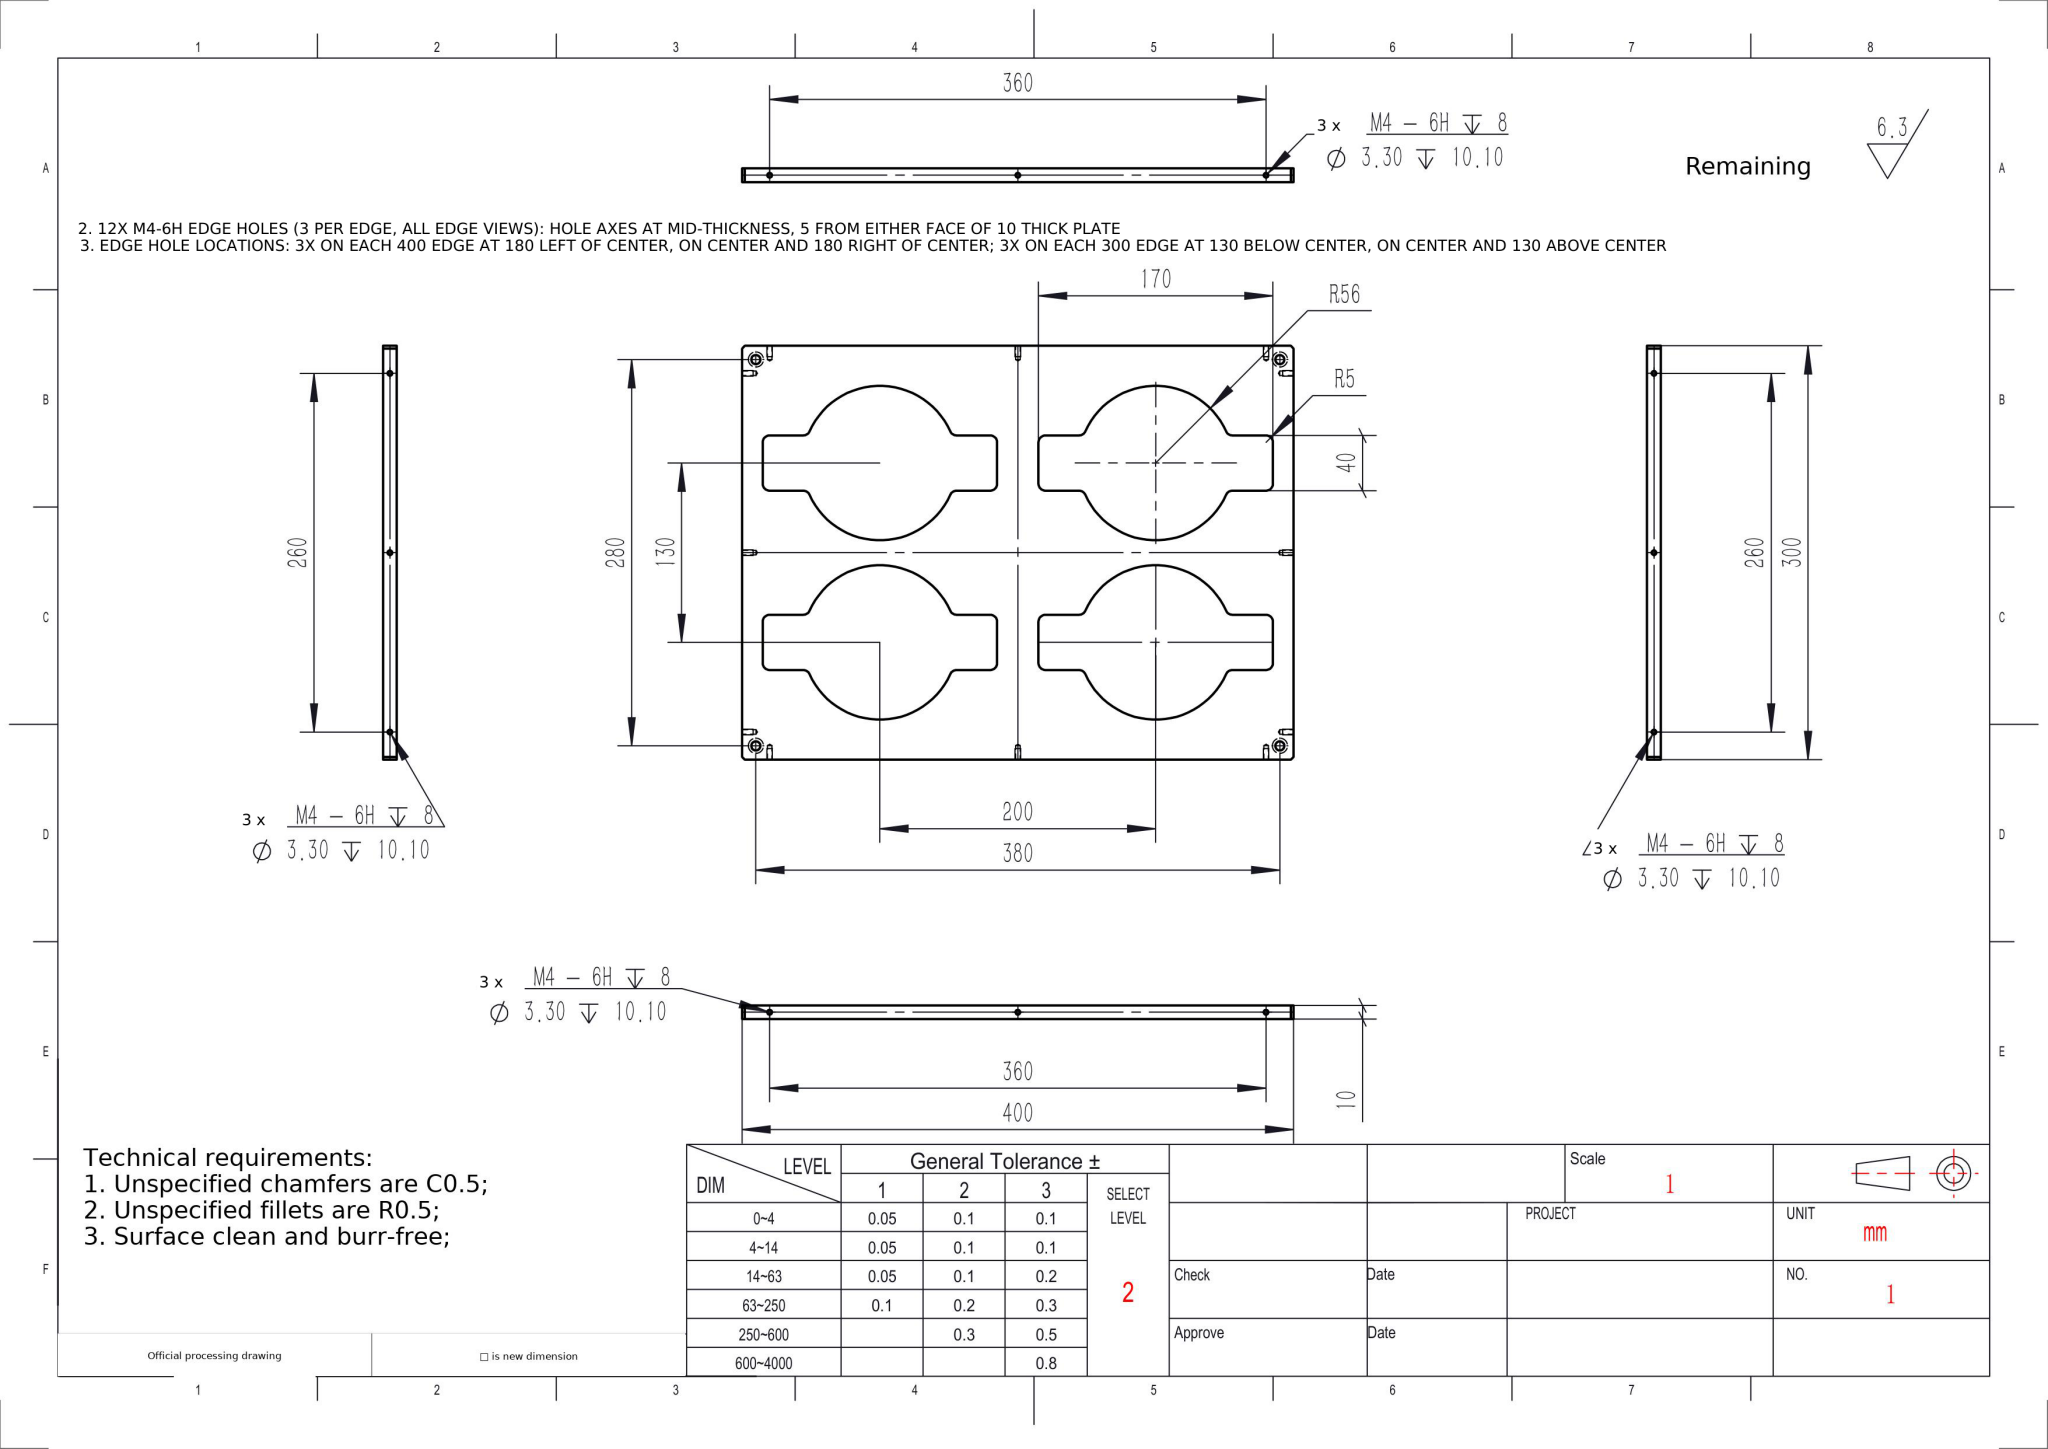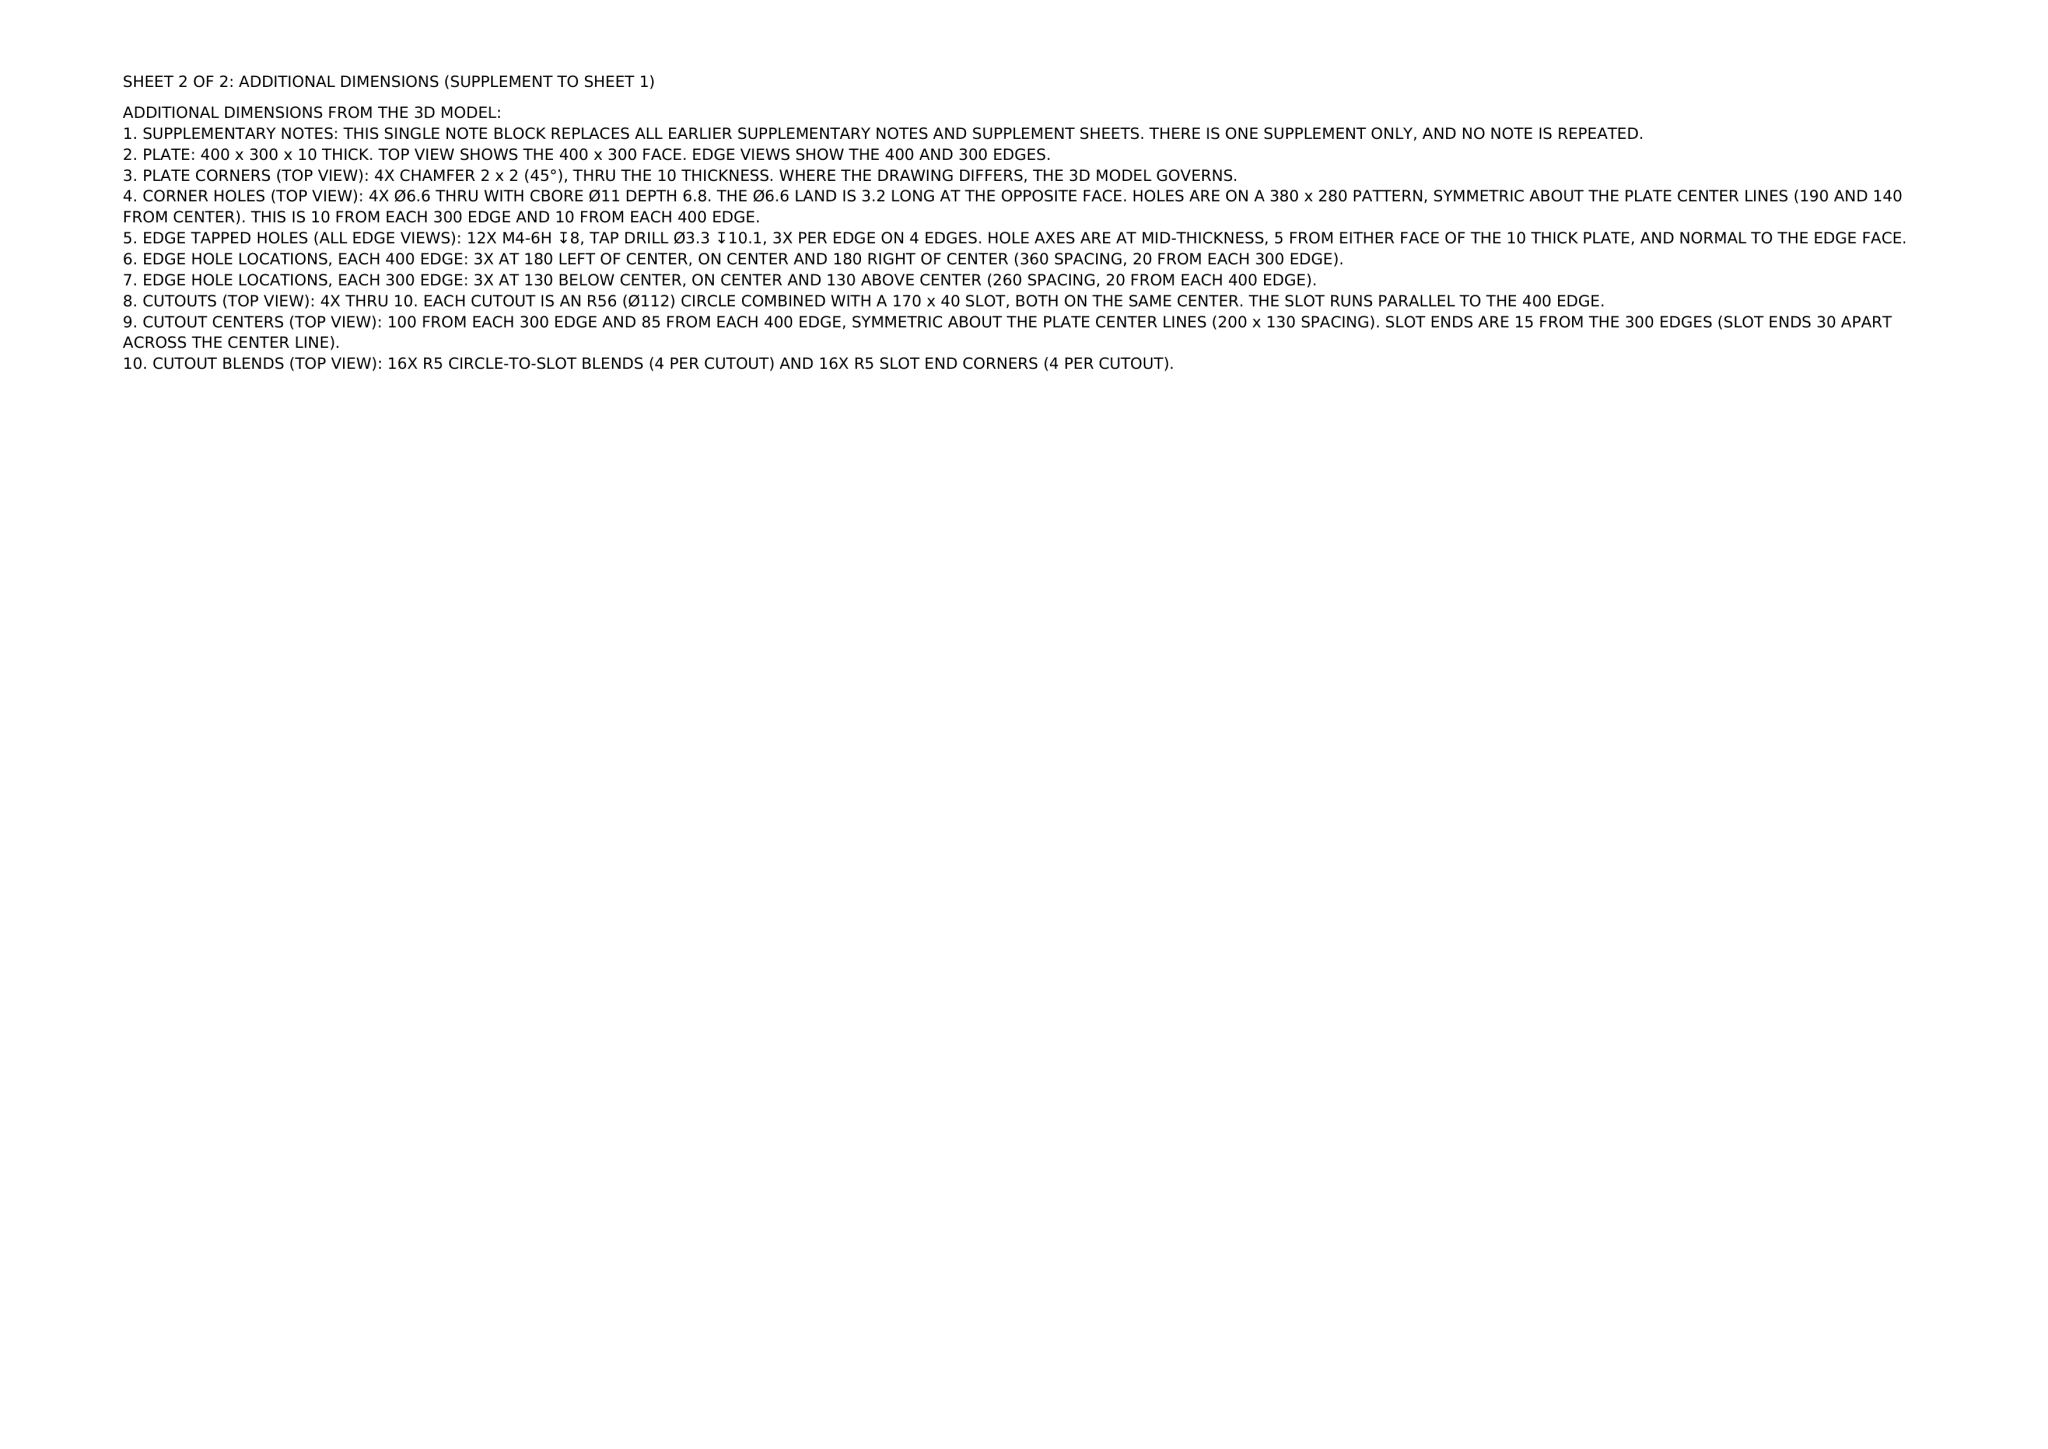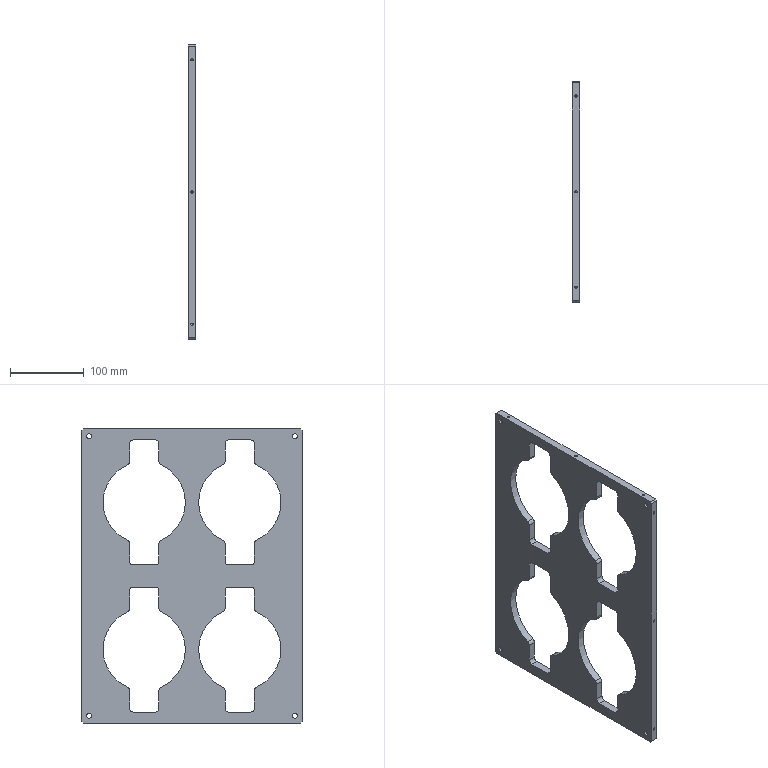Part | NX | mm | 1 solid | 142 faces | box 10 x 300 x 400 mm | volume 705611 mm3 | cylinder 80 | plane 38 | cone 24 | commonest cylinder face diameters 10 x32 3.3 x24 11 x8 6.6 x8 112 x8